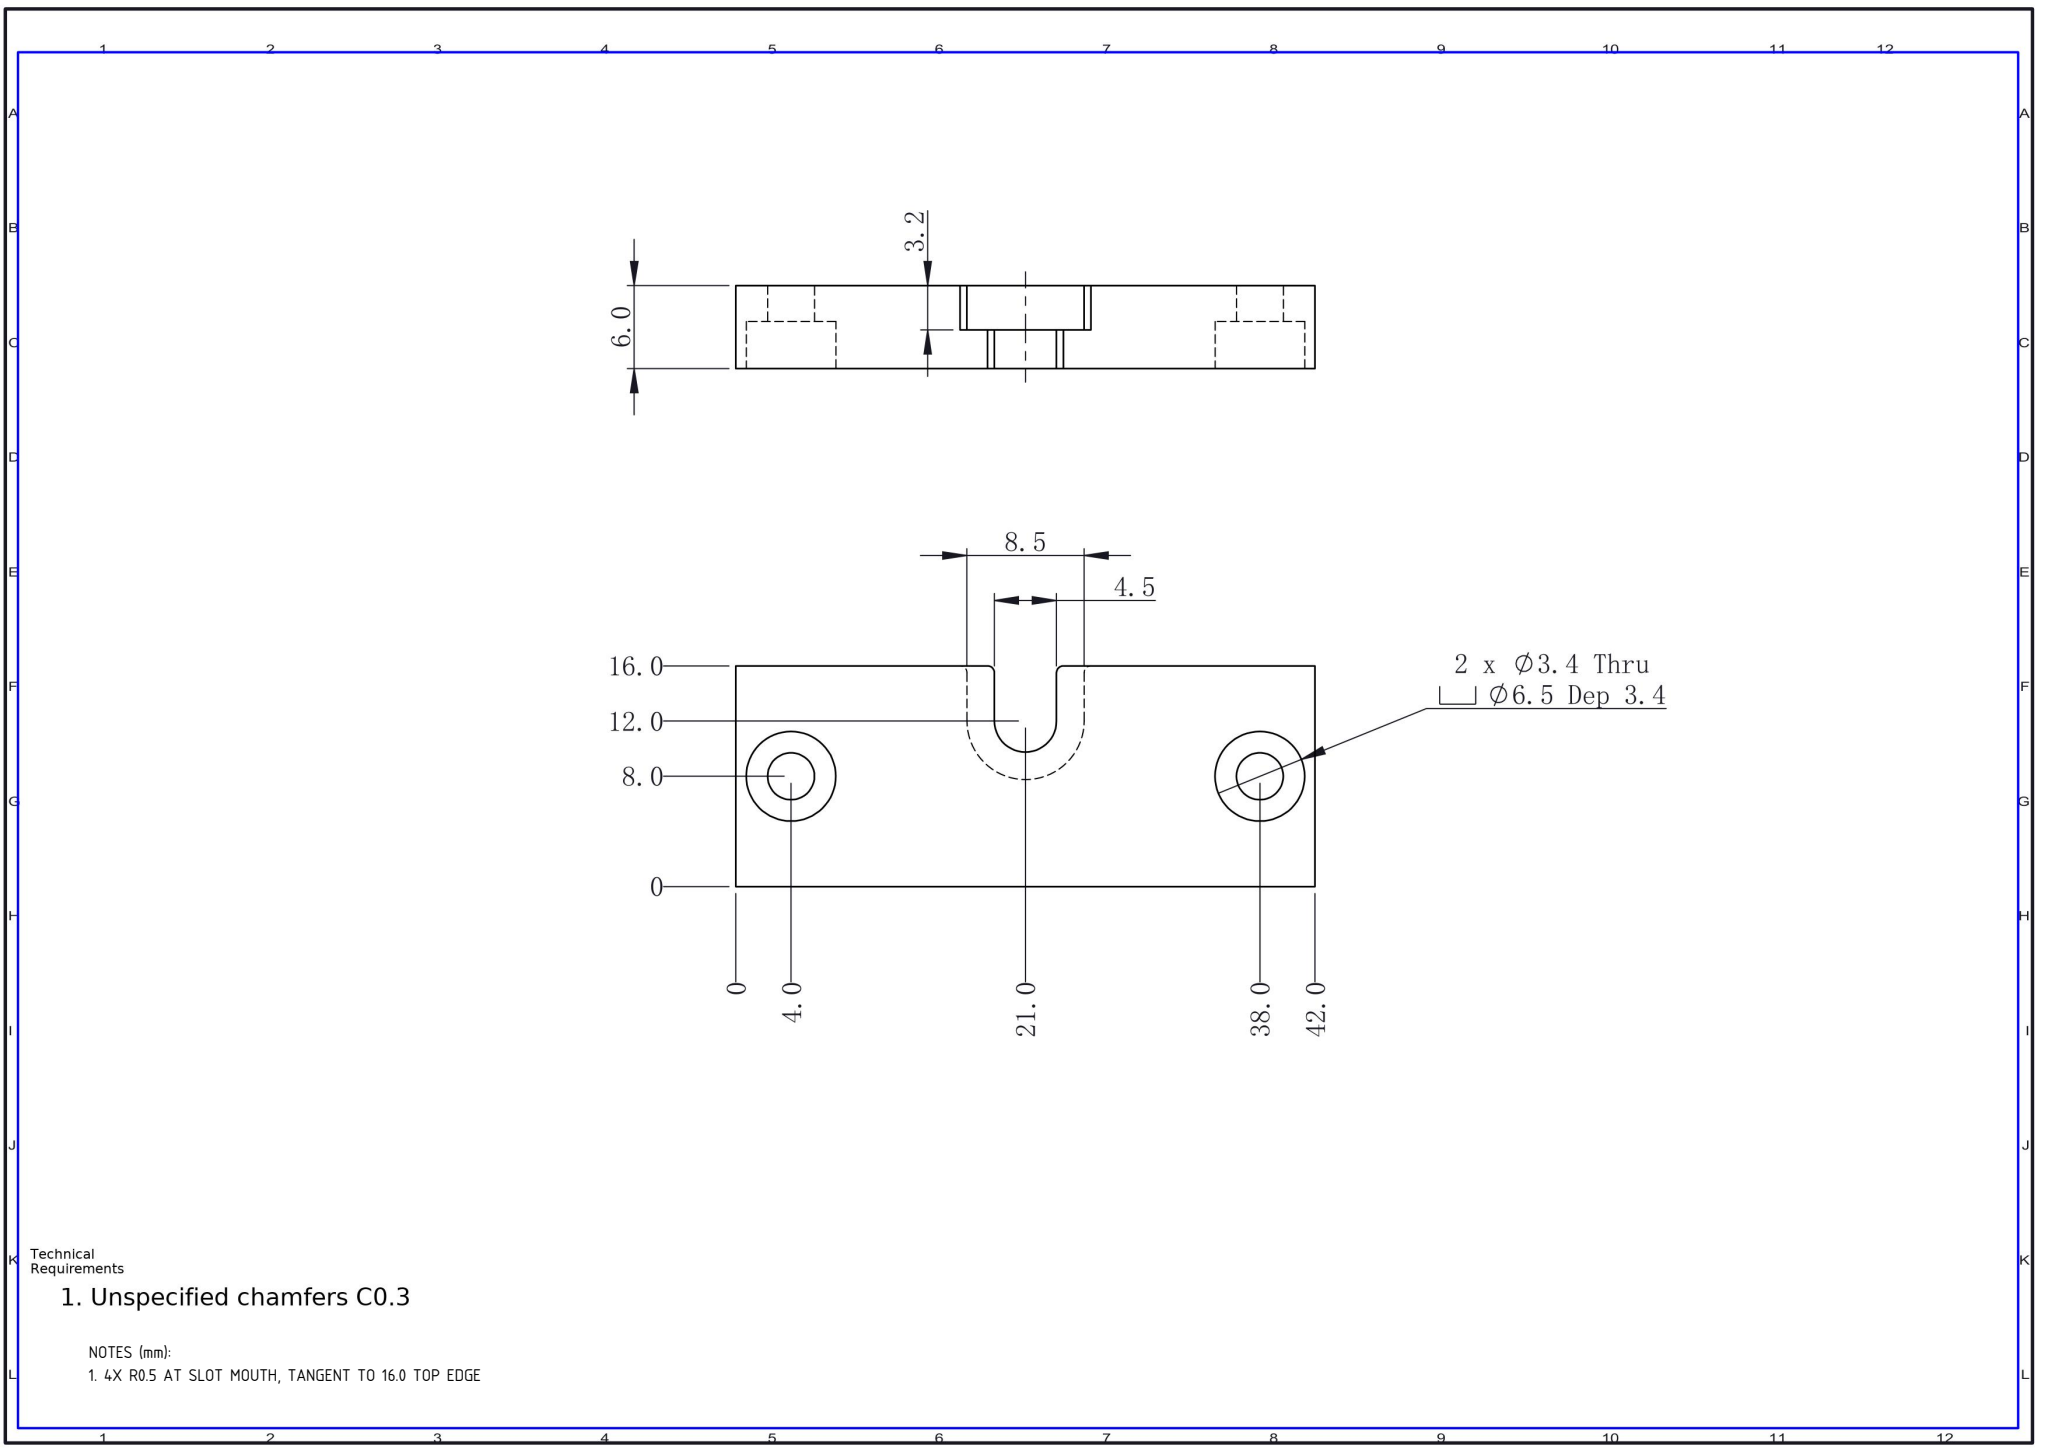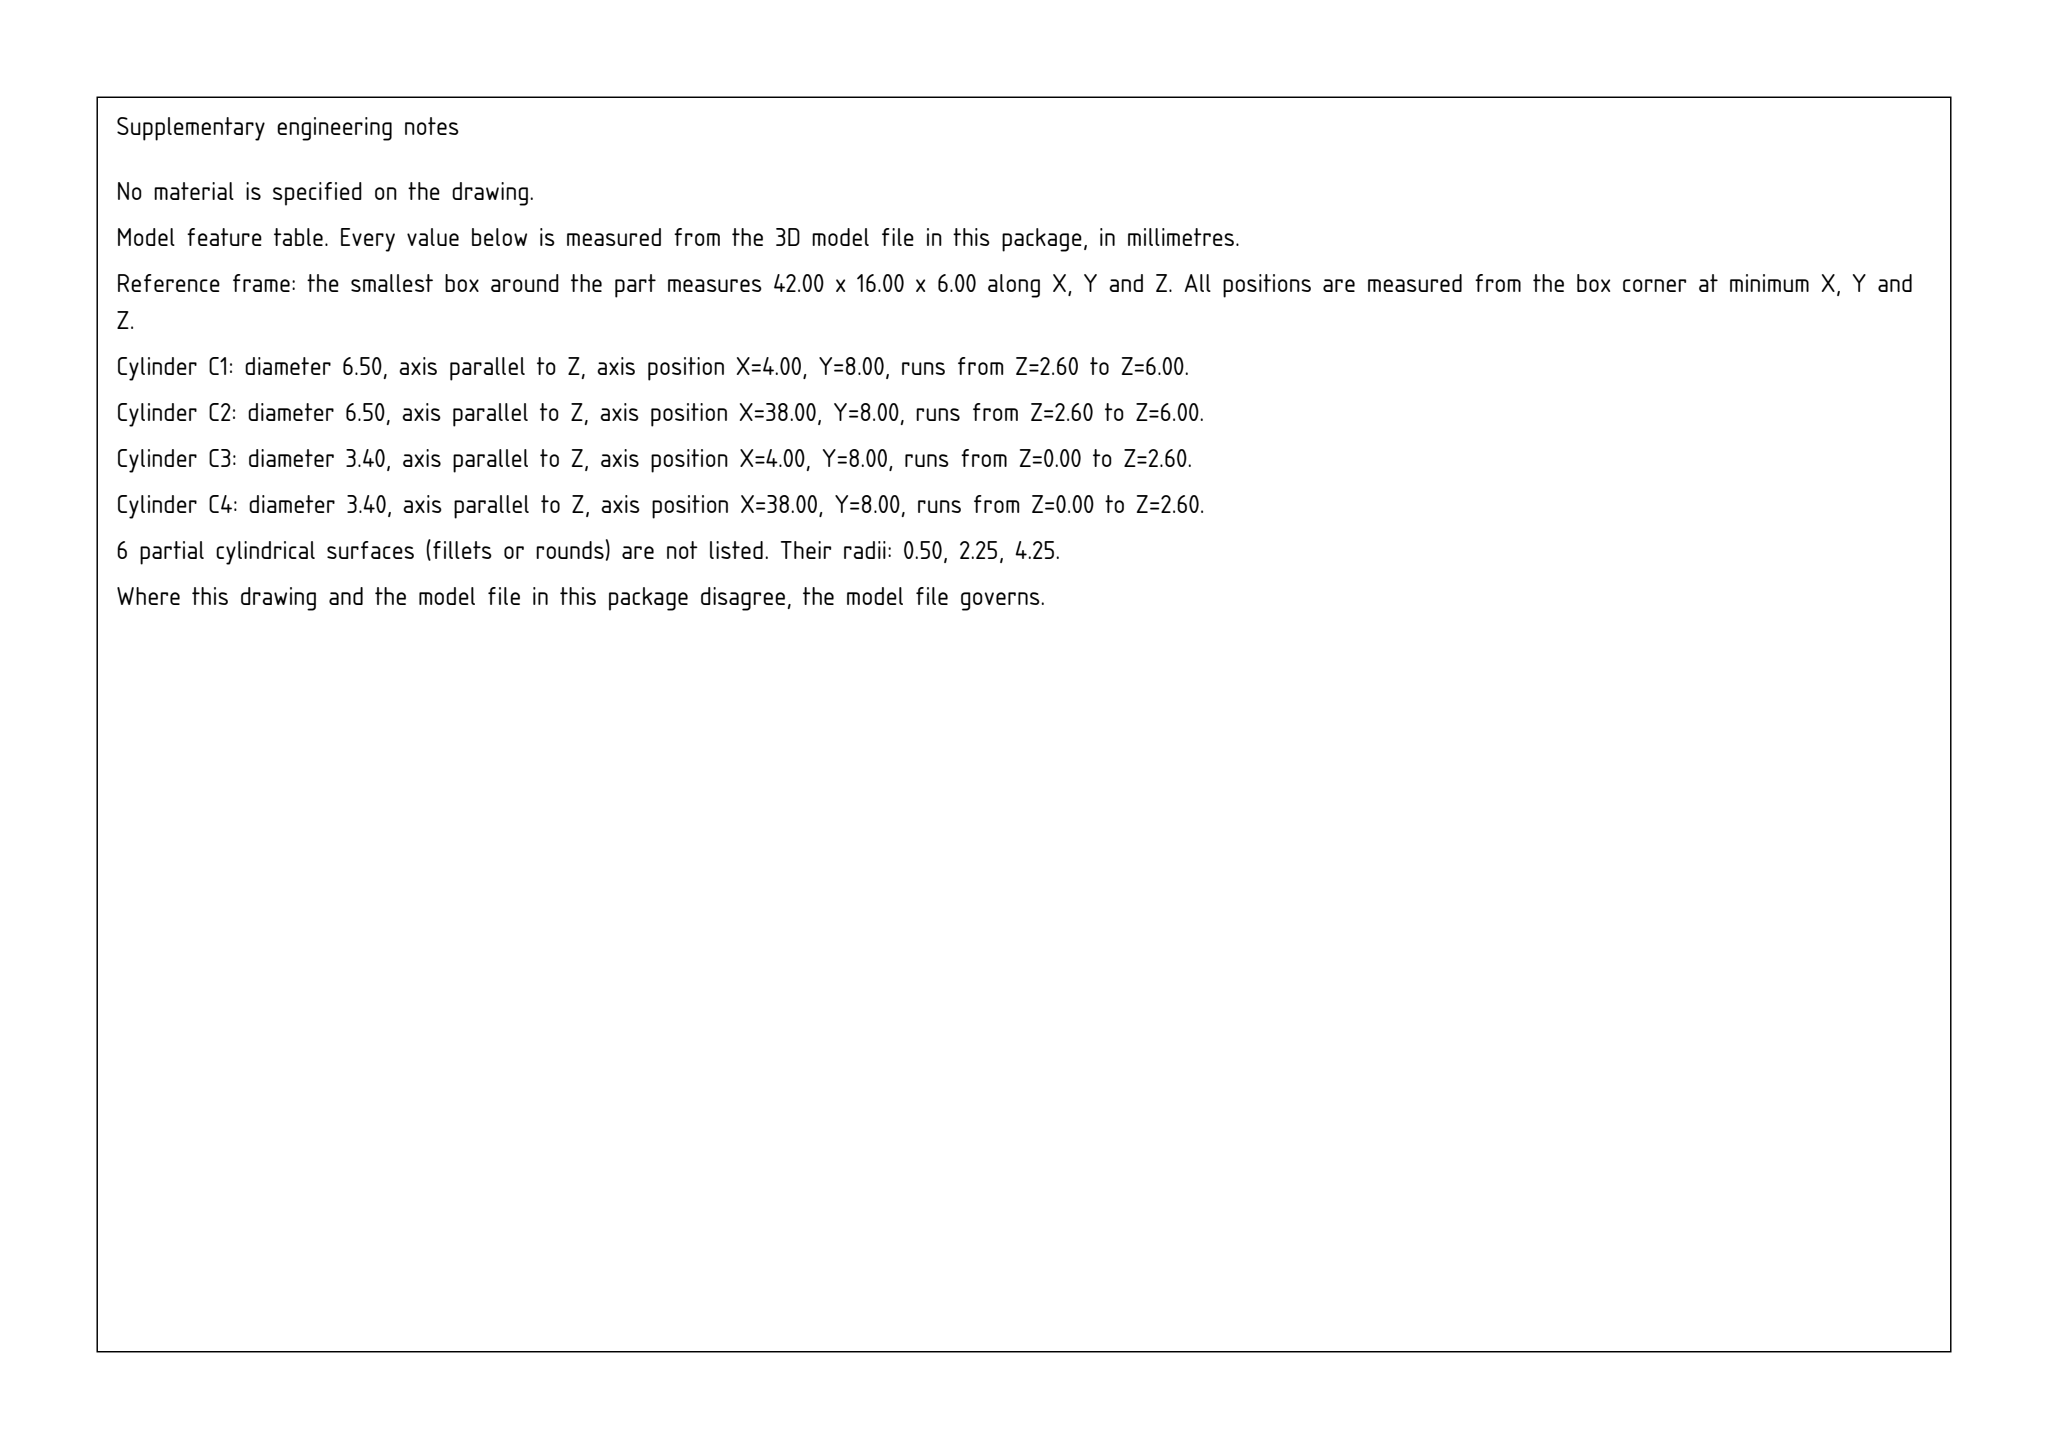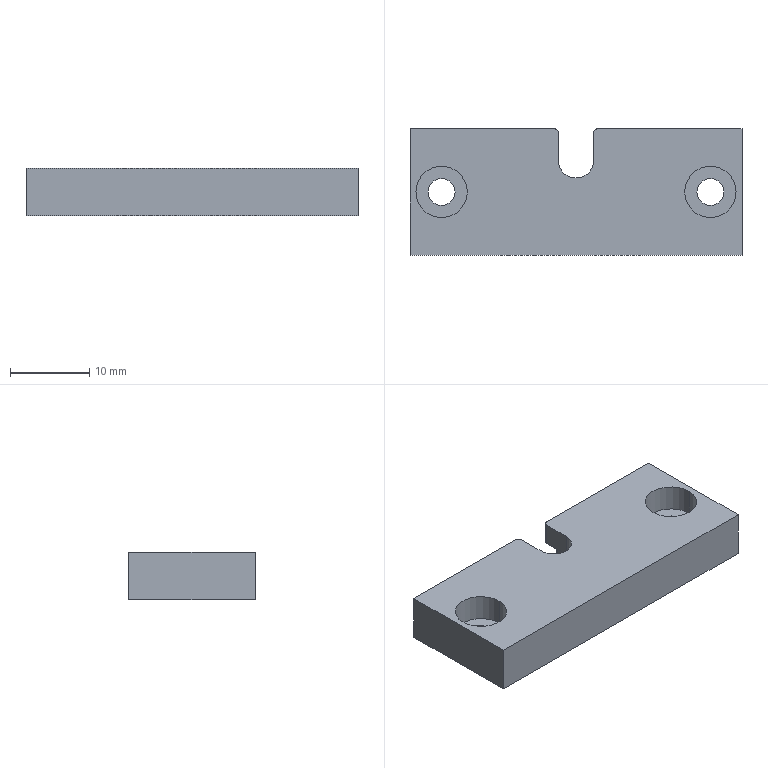Part | SolidWorks | mm | 1 solid | 28 faces | box 42 x 16 x 6 mm | volume 3486 mm3 | cylinder 14 | plane 14 | commonest cylinder face diameters 6.5 x4 3.4 x4 1 x4 8.5 x1 4.5 x1
Drawing notes:
4X R0.5 AT SLOT MOUTH, TANGENT TO 16.0 TOP EDGE | from the solid: Four 1.0 dia z-cylinders at (16.25,15.5),(18.25,15.5),(23.75,15.5),(25.75,15.5) = R0.5, 0.5 from y=16.0 face; slot walls x=16.75/25.25 (8.5 wide) and x=18.75/23.25 (4.5 wide)
build123d program:
from build123d import *

# Parameters (mm, degrees)
SKETCH1_W                                       = 42
SKETCH1_H                                       = 16
BOSS_EXTRUDE1_DEPTH                             = 6
M3_HEX_SOCKET_HEAD_CAP_SCREW_CBORE1_D           = 3.4
M3_HEX_SOCKET_HEAD_CAP_SCREW_CBORE1_CBORE_D     = 6.5
M3_HEX_SOCKET_HEAD_CAP_SCREW_CBORE1_CBORE_DEPTH = 3.4
CUT_EXTRUDE1_DEPTH                              = 3.2
CUT_EXTRUDE2_DEPTH                              = 46.058
FILLET1_R                                       = 0.5


with BuildPart() as part:
    # Sketch1 → Boss-Extrude1 (new body)
    with BuildSketch(Plane.XY):
        with Locations((21, 8)):
            Rectangle(SKETCH1_W, SKETCH1_H)
    extrude(amount=BOSS_EXTRUDE1_DEPTH)

    # M3 Hex Socket Head Cap Screw CBORE1 (through all)
    with Locations(Plane.XY.offset(6)):
        with Locations((4, 8), (38, 8)):
            CounterBoreHole(M3_HEX_SOCKET_HEAD_CAP_SCREW_CBORE1_D / 2, M3_HEX_SOCKET_HEAD_CAP_SCREW_CBORE1_CBORE_D / 2, M3_HEX_SOCKET_HEAD_CAP_SCREW_CBORE1_CBORE_DEPTH)

    # Sketch5 → Cut-Extrude1 (cut)
    with BuildSketch(Plane(origin=(0, 0, 0), x_dir=(-1, 0, 0), z_dir=(0, 0, -1))):
        with BuildLine():
            Line((-16.75, 16), (-16.75, 12))
            ThreePointArc((-16.75, 12), (-21, 7.75), (-25.25, 12))
            Line((-25.25, 12), (-25.25, 16))
            ThreePointArc((-25.25, 16), (-21, 20.25), (-16.75, 16))
        make_face()
    extrude(amount=-CUT_EXTRUDE1_DEPTH, mode=Mode.SUBTRACT)

    # Sketch6 → Cut-Extrude2 (cut, through all)
    with BuildSketch(Plane(origin=(0, 0, 3.2), x_dir=(-1, 0, 0), z_dir=(0, 0, -1))):
        with BuildLine():
            Line((-18.75, 16), (-18.75, 12))
            ThreePointArc((-18.75, 12), (-21, 9.75), (-23.25, 12))
            Line((-23.25, 12), (-23.25, 16))
            ThreePointArc((-23.25, 16), (-21, 18.25), (-18.75, 16))
        make_face()
    extrude(amount=-CUT_EXTRUDE2_DEPTH, mode=Mode.SUBTRACT)

    # Fillet1
    fillet1_edges = [part.edges().sort_by_distance(p)[0] for p in [
        (25.25, 16, 1.6),
        (16.75, 16, 1.6),
        (23.25, 16, 4.6),
        (18.75, 16, 4.6),
    ]]
    fillet(fillet1_edges, radius=FILLET1_R)


solid = part.part